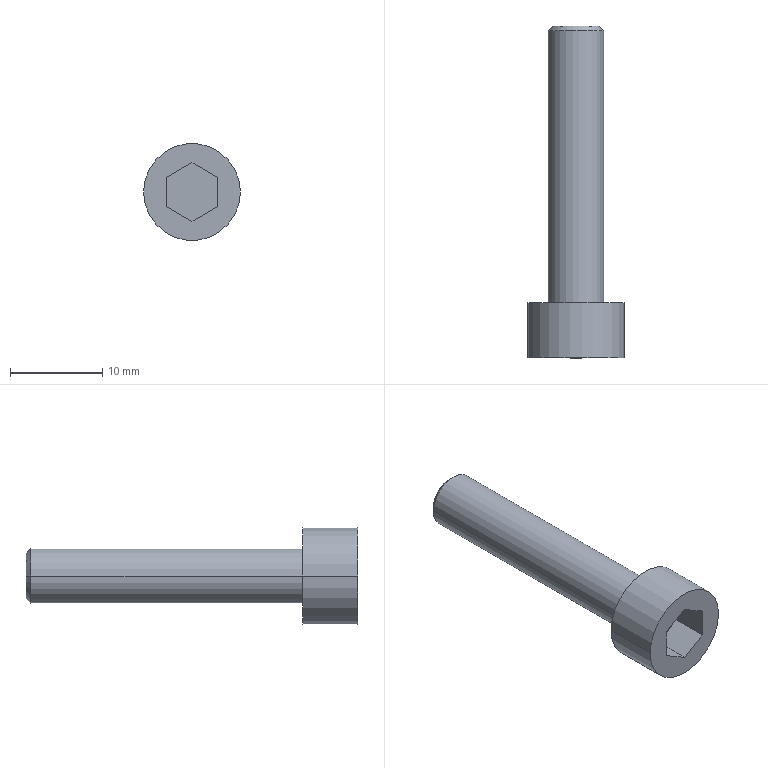Component | SolidWorks | M6x30HexSocketCap-1 | 1 solid | 16 faces | box 10.5 x 36 x 10.5 mm | volume 1261 mm3 | plane 10 | cylinder 4 | cone 2 | commonest cylinder face diameters 6 x2 10.5 x2 | material #45
build123d program:
from build123d import *

# Parameters (mm, degrees)
CUT_EXTRUDE1_DEPTH = 4


with BuildPart() as part:
    # Sketch1 → Revolve1 (revolve)
    with BuildSketch(Plane(origin=(0, 0, 0), x_dir=(1, 0, 0), z_dir=(0, 1, 0)), mode=Mode.PRIVATE) as revolve1_sk:
        Polygon((0, 36), (-5.25, 36), (-5.25, 30), (-3, 30), (-3, 0.5), (-2.5, 0), (0, 0), align=None)
    revolve(revolve1_sk.sketch.rotate(Axis((0, 0, 0), (0, 0, -1)), 180), axis=Axis((0, 0, 0), (0, 0, -1)))

    # Sketch2 → Cut-Extrude1 (cut)
    with BuildSketch(Plane(origin=(0, 0, -36), x_dir=(-1, 0, 0), z_dir=(0, 0, -1))):
        Polygon((0, 3.175), (-2.75, 1.588), (-2.75, -1.588), (0, -3.175), (2.75, -1.588), (2.75, 1.588), align=None)
    extrude(amount=-CUT_EXTRUDE1_DEPTH, mode=Mode.SUBTRACT)


solid = part.part

# Placed as in the assembly
solid = solid.moved(Location((-63, 340.7, 7.5), (-90, 0, 0)))
STEP:
#1=COLOUR_RGB('',0.7922,0.8196,0.9333);
#2=FILL_AREA_STYLE_COLOUR('',#1);
#3=FILL_AREA_STYLE('',(#2));
#4=SURFACE_STYLE_FILL_AREA(#3);
#5=SURFACE_SIDE_STYLE('',(#4));
#6=SURFACE_STYLE_USAGE(.BOTH.,#5);
#7=PRESENTATION_STYLE_ASSIGNMENT((#6));
#8=CARTESIAN_POINT('',(-2.382,13.413,0.2953));
#9=VERTEX_POINT('',#8);
#10=CARTESIAN_POINT('',(-2.579,13.413,0.2953));
#11=VERTEX_POINT('',#10);
#12=CARTESIAN_POINT('',(-2.48,13.413,0.2953));
#13=DIRECTION('',(0.,1.,-0.));
#14=DIRECTION('',(1.,0.,0.));
#15=AXIS2_PLACEMENT_3D('',#12,#13,#14);
#16=CIRCLE('',#15,0.09843);
#17=EDGE_CURVE('',#9,#11,#16,.T.);
#18=ORIENTED_EDGE('',*,*,#17,.F.);
#19=CARTESIAN_POINT('',(-2.362,13.394,0.2953));
#20=VERTEX_POINT('',#19);
#21=CARTESIAN_POINT('',(-2.362,13.394,0.2953));
#22=DIRECTION('',(0.7071,-0.7071,-0.));
#23=VECTOR('',#22,39.37);
#24=LINE('',#21,#23);
#25=EDGE_CURVE('',#9,#20,#24,.T.);
#26=ORIENTED_EDGE('',*,*,#25,.T.);
#27=CARTESIAN_POINT('',(-2.598,13.394,0.2953));
#28=VERTEX_POINT('',#27);
#29=CARTESIAN_POINT('',(-2.48,13.394,0.2953));
#30=DIRECTION('',(0.,1.,-0.));
#31=DIRECTION('',(1.,0.,0.));
#32=AXIS2_PLACEMENT_3D('',#29,#30,#31);
#33=CIRCLE('',#32,0.1181);
#34=EDGE_CURVE('',#20,#28,#33,.T.);
#35=ORIENTED_EDGE('',*,*,#34,.T.);
#36=CARTESIAN_POINT('',(-2.598,13.394,0.2953));
#37=DIRECTION('',(-0.7071,-0.7071,0.));
#38=VECTOR('',#37,39.37);
#39=LINE('',#36,#38);
#40=EDGE_CURVE('',#11,#28,#39,.T.);
#41=ORIENTED_EDGE('',*,*,#40,.F.);
#42=EDGE_LOOP('',(#18,#26,#35,#41));
#43=FACE_OUTER_BOUND('',#42,.T.);
#44=CARTESIAN_POINT('',(-2.48,13.394,0.2953));
#45=DIRECTION('',(-0.,-1.,0.));
#46=DIRECTION('',(-1.,0.,0.));
#47=AXIS2_PLACEMENT_3D('',#44,#45,#46);
#48=CONICAL_SURFACE('',#47,0.1181,0.7854);
#49=ADVANCED_FACE('',(#43),#48,.T.);
#50=CARTESIAN_POINT('',(-2.362,12.232,0.2953));
#51=VERTEX_POINT('',#50);
#52=CARTESIAN_POINT('',(-2.598,12.232,0.2953));
#53=VERTEX_POINT('',#52);
#54=CARTESIAN_POINT('',(-2.48,12.232,0.2953));
#55=DIRECTION('',(0.,1.,-0.));
#56=DIRECTION('',(1.,0.,0.));
#57=AXIS2_PLACEMENT_3D('',#54,#55,#56);
#58=CIRCLE('',#57,0.1181);
#59=EDGE_CURVE('',#51,#53,#58,.T.);
#60=ORIENTED_EDGE('',*,*,#59,.T.);
#61=CARTESIAN_POINT('',(-2.598,13.413,0.2953));
#62=DIRECTION('',(0.,1.,-0.));
#63=VECTOR('',#62,39.37);
#64=LINE('',#61,#63);
#65=EDGE_CURVE('',#53,#28,#64,.T.);
#66=ORIENTED_EDGE('',*,*,#65,.T.);
#67=ORIENTED_EDGE('',*,*,#34,.F.);
#68=CARTESIAN_POINT('',(-2.362,13.413,0.2953));
#69=DIRECTION('',(0.,1.,-0.));
#70=VECTOR('',#69,39.37);
#71=LINE('',#68,#70);
#72=EDGE_CURVE('',#51,#20,#71,.T.);
#73=ORIENTED_EDGE('',*,*,#72,.F.);
#74=EDGE_LOOP('',(#60,#66,#67,#73));
#75=FACE_OUTER_BOUND('',#74,.T.);
#76=CARTESIAN_POINT('',(-2.48,13.413,0.2953));
#77=DIRECTION('',(0.,1.,-0.));
#78=DIRECTION('',(1.,0.,0.));
#79=AXIS2_PLACEMENT_3D('',#76,#77,#78);
#80=CYLINDRICAL_SURFACE('',#79,0.1181);
#81=ADVANCED_FACE('',(#75),#80,.T.);
#82=CARTESIAN_POINT('',(-2.274,11.996,0.2953));
#83=VERTEX_POINT('',#82);
#84=CARTESIAN_POINT('',(-2.687,11.996,0.2953));
#85=VERTEX_POINT('',#84);
#86=CARTESIAN_POINT('',(-2.48,11.996,0.2953));
#87=DIRECTION('',(0.,1.,-0.));
#88=DIRECTION('',(1.,0.,0.));
#89=AXIS2_PLACEMENT_3D('',#86,#87,#88);
#90=CIRCLE('',#89,0.2067);
#91=EDGE_CURVE('',#83,#85,#90,.T.);
#92=ORIENTED_EDGE('',*,*,#91,.T.);
#93=CARTESIAN_POINT('',(-2.687,12.232,0.2953));
#94=VERTEX_POINT('',#93);
#95=CARTESIAN_POINT('',(-2.687,13.413,0.2953));
#96=DIRECTION('',(0.,1.,-0.));
#97=VECTOR('',#96,39.37);
#98=LINE('',#95,#97);
#99=EDGE_CURVE('',#85,#94,#98,.T.);
#100=ORIENTED_EDGE('',*,*,#99,.T.);
#101=CARTESIAN_POINT('',(-2.274,12.232,0.2953));
#102=VERTEX_POINT('',#101);
#103=CARTESIAN_POINT('',(-2.48,12.232,0.2953));
#104=DIRECTION('',(0.,1.,-0.));
#105=DIRECTION('',(1.,0.,0.));
#106=AXIS2_PLACEMENT_3D('',#103,#104,#105);
#107=CIRCLE('',#106,0.2067);
#108=EDGE_CURVE('',#102,#94,#107,.T.);
#109=ORIENTED_EDGE('',*,*,#108,.F.);
#110=CARTESIAN_POINT('',(-2.274,13.413,0.2953));
#111=DIRECTION('',(0.,1.,-0.));
#112=VECTOR('',#111,39.37);
#113=LINE('',#110,#112);
#114=EDGE_CURVE('',#83,#102,#113,.T.);
#115=ORIENTED_EDGE('',*,*,#114,.F.);
#116=EDGE_LOOP('',(#92,#100,#109,#115));
#117=FACE_OUTER_BOUND('',#116,.T.);
#118=CARTESIAN_POINT('',(-2.48,13.413,0.2953));
#119=DIRECTION('',(0.,1.,-0.));
#120=DIRECTION('',(1.,0.,0.));
#121=AXIS2_PLACEMENT_3D('',#118,#119,#120);
#122=CYLINDRICAL_SURFACE('',#121,0.2067);
#123=ADVANCED_FACE('',(#117),#122,.T.);
#124=CARTESIAN_POINT('',(-2.48,11.996,0.1703));
#125=VERTEX_POINT('',#124);
#126=CARTESIAN_POINT('',(-2.372,11.996,0.2328));
#127=VERTEX_POINT('',#126);
#128=CARTESIAN_POINT('',(-2.48,11.996,0.1703));
#129=DIRECTION('',(0.866,0.,0.5));
#130=VECTOR('',#129,39.37);
#131=LINE('',#128,#130);
#132=EDGE_CURVE('',#125,#127,#131,.T.);
#133=ORIENTED_EDGE('',*,*,#132,.F.);
#134=CARTESIAN_POINT('',(-2.589,11.996,0.2328));
#135=VERTEX_POINT('',#134);
#136=CARTESIAN_POINT('',(-2.589,11.996,0.2328));
#137=DIRECTION('',(0.866,-0.,-0.5));
#138=VECTOR('',#137,39.37);
#139=LINE('',#136,#138);
#140=EDGE_CURVE('',#135,#125,#139,.T.);
#141=ORIENTED_EDGE('',*,*,#140,.F.);
#142=CARTESIAN_POINT('',(-2.589,11.996,0.3578));
#143=VERTEX_POINT('',#142);
#144=CARTESIAN_POINT('',(-2.589,11.996,0.3578));
#145=DIRECTION('',(-0.,-0.,-1.));
#146=VECTOR('',#145,39.37);
#147=LINE('',#144,#146);
#148=EDGE_CURVE('',#143,#135,#147,.T.);
#149=ORIENTED_EDGE('',*,*,#148,.F.);
#150=CARTESIAN_POINT('',(-2.48,11.996,0.4203));
#151=VERTEX_POINT('',#150);
#152=CARTESIAN_POINT('',(-2.48,11.996,0.4203));
#153=DIRECTION('',(-0.866,-0.,-0.5));
#154=VECTOR('',#153,39.37);
#155=LINE('',#152,#154);
#156=EDGE_CURVE('',#151,#143,#155,.T.);
#157=ORIENTED_EDGE('',*,*,#156,.F.);
#158=CARTESIAN_POINT('',(-2.372,11.996,0.3578));
#159=VERTEX_POINT('',#158);
#160=CARTESIAN_POINT('',(-2.372,11.996,0.3578));
#161=DIRECTION('',(-0.866,0.,0.5));
#162=VECTOR('',#161,39.37);
#163=LINE('',#160,#162);
#164=EDGE_CURVE('',#159,#151,#163,.T.);
#165=ORIENTED_EDGE('',*,*,#164,.F.);
#166=CARTESIAN_POINT('',(-2.372,11.996,0.2328));
#167=DIRECTION('',(0.,0.,1.));
#168=VECTOR('',#167,39.37);
#169=LINE('',#166,#168);
#170=EDGE_CURVE('',#127,#159,#169,.T.);
#171=ORIENTED_EDGE('',*,*,#170,.F.);
#172=EDGE_LOOP('',(#133,#141,#149,#157,#165,#171));
#173=FACE_BOUND('',#172,.T.);
#174=ORIENTED_EDGE('',*,*,#91,.F.);
#175=CARTESIAN_POINT('',(-2.48,11.996,0.2953));
#176=DIRECTION('',(0.,1.,-0.));
#177=DIRECTION('',(1.,0.,0.));
#178=AXIS2_PLACEMENT_3D('',#175,#176,#177);
#179=CIRCLE('',#178,0.2067);
#180=EDGE_CURVE('',#85,#83,#179,.T.);
#181=ORIENTED_EDGE('',*,*,#180,.F.);
#182=EDGE_LOOP('',(#174,#181));
#183=FACE_OUTER_BOUND('',#182,.T.);
#184=CARTESIAN_POINT('',(-2.48,11.996,0.2953));
#185=DIRECTION('',(0.,1.,-0.));
#186=DIRECTION('',(1.,-0.,-0.));
#187=AXIS2_PLACEMENT_3D('',#184,#185,#186);
#188=PLANE('',#187);
#189=ADVANCED_FACE('',(#173,#183),#188,.F.);
#190=ORIENTED_EDGE('',*,*,#99,.F.);
#191=ORIENTED_EDGE('',*,*,#180,.T.);
#192=ORIENTED_EDGE('',*,*,#114,.T.);
#193=CARTESIAN_POINT('',(-2.48,12.232,0.2953));
#194=DIRECTION('',(0.,1.,-0.));
#195=DIRECTION('',(1.,0.,0.));
#196=AXIS2_PLACEMENT_3D('',#193,#194,#195);
#197=CIRCLE('',#196,0.2067);
#198=EDGE_CURVE('',#94,#102,#197,.T.);
#199=ORIENTED_EDGE('',*,*,#198,.F.);
#200=EDGE_LOOP('',(#190,#191,#192,#199));
#201=FACE_OUTER_BOUND('',#200,.T.);
#202=CARTESIAN_POINT('',(-2.48,13.413,0.2953));
#203=DIRECTION('',(0.,1.,-0.));
#204=DIRECTION('',(1.,0.,0.));
#205=AXIS2_PLACEMENT_3D('',#202,#203,#204);
#206=CYLINDRICAL_SURFACE('',#205,0.2067);
#207=ADVANCED_FACE('',(#201),#206,.T.);
#208=ORIENTED_EDGE('',*,*,#59,.F.);
#209=CARTESIAN_POINT('',(-2.48,12.232,0.2953));
#210=DIRECTION('',(0.,1.,-0.));
#211=DIRECTION('',(1.,0.,0.));
#212=AXIS2_PLACEMENT_3D('',#209,#210,#211);
#213=CIRCLE('',#212,0.1181);
#214=EDGE_CURVE('',#53,#51,#213,.T.);
#215=ORIENTED_EDGE('',*,*,#214,.F.);
#216=EDGE_LOOP('',(#208,#215));
#217=FACE_BOUND('',#216,.T.);
#218=ORIENTED_EDGE('',*,*,#108,.T.);
#219=ORIENTED_EDGE('',*,*,#198,.T.);
#220=EDGE_LOOP('',(#218,#219));
#221=FACE_OUTER_BOUND('',#220,.T.);
#222=CARTESIAN_POINT('',(-2.687,12.232,0.2953));
#223=DIRECTION('',(-0.,-1.,0.));
#224=DIRECTION('',(-1.,0.,0.));
#225=AXIS2_PLACEMENT_3D('',#222,#223,#224);
#226=PLANE('',#225);
#227=ADVANCED_FACE('',(#217,#221),#226,.F.);
#228=ORIENTED_EDGE('',*,*,#65,.F.);
#229=ORIENTED_EDGE('',*,*,#214,.T.);
#230=ORIENTED_EDGE('',*,*,#72,.T.);
#231=CARTESIAN_POINT('',(-2.48,13.394,0.2953));
#232=DIRECTION('',(0.,1.,-0.));
#233=DIRECTION('',(1.,0.,0.));
#234=AXIS2_PLACEMENT_3D('',#231,#232,#233);
#235=CIRCLE('',#234,0.1181);
#236=EDGE_CURVE('',#28,#20,#235,.T.);
#237=ORIENTED_EDGE('',*,*,#236,.F.);
#238=EDGE_LOOP('',(#228,#229,#230,#237));
#239=FACE_OUTER_BOUND('',#238,.T.);
#240=CARTESIAN_POINT('',(-2.48,13.413,0.2953));
#241=DIRECTION('',(0.,1.,-0.));
#242=DIRECTION('',(1.,0.,0.));
#243=AXIS2_PLACEMENT_3D('',#240,#241,#242);
#244=CYLINDRICAL_SURFACE('',#243,0.1181);
#245=ADVANCED_FACE('',(#239),#244,.T.);
#246=ORIENTED_EDGE('',*,*,#25,.F.);
#247=CARTESIAN_POINT('',(-2.48,13.413,0.2953));
#248=DIRECTION('',(0.,1.,-0.));
#249=DIRECTION('',(1.,0.,0.));
#250=AXIS2_PLACEMENT_3D('',#247,#248,#249);
#251=CIRCLE('',#250,0.09843);
#252=EDGE_CURVE('',#11,#9,#251,.T.);
#253=ORIENTED_EDGE('',*,*,#252,.F.);
#254=ORIENTED_EDGE('',*,*,#40,.T.);
#255=ORIENTED_EDGE('',*,*,#236,.T.);
#256=EDGE_LOOP('',(#246,#253,#254,#255));
#257=FACE_OUTER_BOUND('',#256,.T.);
#258=CARTESIAN_POINT('',(-2.48,13.394,0.2953));
#259=DIRECTION('',(-0.,-1.,0.));
#260=DIRECTION('',(-1.,0.,0.));
#261=AXIS2_PLACEMENT_3D('',#258,#259,#260);
#262=CONICAL_SURFACE('',#261,0.1181,0.7854);
#263=ADVANCED_FACE('',(#257),#262,.T.);
#264=ORIENTED_EDGE('',*,*,#252,.T.);
#265=ORIENTED_EDGE('',*,*,#17,.T.);
#266=EDGE_LOOP('',(#264,#265));
#267=FACE_OUTER_BOUND('',#266,.T.);
#268=CARTESIAN_POINT('',(-2.579,13.413,0.2953));
#269=DIRECTION('',(-0.,-1.,0.));
#270=DIRECTION('',(-1.,0.,0.));
#271=AXIS2_PLACEMENT_3D('',#268,#269,#270);
#272=PLANE('',#271);
#273=ADVANCED_FACE('',(#267),#272,.F.);
#274=ORIENTED_EDGE('',*,*,#140,.T.);
#275=CARTESIAN_POINT('',(-2.48,12.154,0.1703));
#276=VERTEX_POINT('',#275);
#277=CARTESIAN_POINT('',(-2.48,12.154,0.1703));
#278=DIRECTION('',(-0.,-1.,0.));
#279=VECTOR('',#278,39.37);
#280=LINE('',#277,#279);
#281=EDGE_CURVE('',#276,#125,#280,.T.);
#282=ORIENTED_EDGE('',*,*,#281,.F.);
#283=CARTESIAN_POINT('',(-2.589,12.154,0.2328));
#284=VERTEX_POINT('',#283);
#285=CARTESIAN_POINT('',(-2.589,12.154,0.2328));
#286=DIRECTION('',(0.866,-0.,-0.5));
#287=VECTOR('',#286,39.37);
#288=LINE('',#285,#287);
#289=EDGE_CURVE('',#284,#276,#288,.T.);
#290=ORIENTED_EDGE('',*,*,#289,.F.);
#291=CARTESIAN_POINT('',(-2.589,12.154,0.2328));
#292=DIRECTION('',(-0.,-1.,0.));
#293=VECTOR('',#292,39.37);
#294=LINE('',#291,#293);
#295=EDGE_CURVE('',#284,#135,#294,.T.);
#296=ORIENTED_EDGE('',*,*,#295,.T.);
#297=EDGE_LOOP('',(#274,#282,#290,#296));
#298=FACE_OUTER_BOUND('',#297,.T.);
#299=CARTESIAN_POINT('',(-2.589,12.154,0.2328));
#300=DIRECTION('',(-0.5,-0.,-0.866));
#301=DIRECTION('',(-0.866,0.,0.5));
#302=AXIS2_PLACEMENT_3D('',#299,#300,#301);
#303=PLANE('',#302);
#304=ADVANCED_FACE('',(#298),#303,.F.);
#305=ORIENTED_EDGE('',*,*,#148,.T.);
#306=ORIENTED_EDGE('',*,*,#295,.F.);
#307=CARTESIAN_POINT('',(-2.589,12.154,0.3578));
#308=VERTEX_POINT('',#307);
#309=CARTESIAN_POINT('',(-2.589,12.154,0.3578));
#310=DIRECTION('',(-0.,-0.,-1.));
#311=VECTOR('',#310,39.37);
#312=LINE('',#309,#311);
#313=EDGE_CURVE('',#308,#284,#312,.T.);
#314=ORIENTED_EDGE('',*,*,#313,.F.);
#315=CARTESIAN_POINT('',(-2.589,12.154,0.3578));
#316=DIRECTION('',(-0.,-1.,0.));
#317=VECTOR('',#316,39.37);
#318=LINE('',#315,#317);
#319=EDGE_CURVE('',#308,#143,#318,.T.);
#320=ORIENTED_EDGE('',*,*,#319,.T.);
#321=EDGE_LOOP('',(#305,#306,#314,#320));
#322=FACE_OUTER_BOUND('',#321,.T.);
#323=CARTESIAN_POINT('',(-2.589,12.154,0.3578));
#324=DIRECTION('',(-1.,0.,0.));
#325=DIRECTION('',(0.,1.,-0.));
#326=AXIS2_PLACEMENT_3D('',#323,#324,#325);
#327=PLANE('',#326);
#328=ADVANCED_FACE('',(#322),#327,.F.);
#329=ORIENTED_EDGE('',*,*,#156,.T.);
#330=ORIENTED_EDGE('',*,*,#319,.F.);
#331=CARTESIAN_POINT('',(-2.48,12.154,0.4203));
#332=VERTEX_POINT('',#331);
#333=CARTESIAN_POINT('',(-2.48,12.154,0.4203));
#334=DIRECTION('',(-0.866,-0.,-0.5));
#335=VECTOR('',#334,39.37);
#336=LINE('',#333,#335);
#337=EDGE_CURVE('',#332,#308,#336,.T.);
#338=ORIENTED_EDGE('',*,*,#337,.F.);
#339=CARTESIAN_POINT('',(-2.48,12.154,0.4203));
#340=DIRECTION('',(-0.,-1.,0.));
#341=VECTOR('',#340,39.37);
#342=LINE('',#339,#341);
#343=EDGE_CURVE('',#332,#151,#342,.T.);
#344=ORIENTED_EDGE('',*,*,#343,.T.);
#345=EDGE_LOOP('',(#329,#330,#338,#344));
#346=FACE_OUTER_BOUND('',#345,.T.);
#347=CARTESIAN_POINT('',(-2.48,12.154,0.4203));
#348=DIRECTION('',(-0.5,0.,0.866));
#349=DIRECTION('',(0.866,0.,0.5));
#350=AXIS2_PLACEMENT_3D('',#347,#348,#349);
#351=PLANE('',#350);
#352=ADVANCED_FACE('',(#346),#351,.F.);
#353=ORIENTED_EDGE('',*,*,#164,.T.);
#354=ORIENTED_EDGE('',*,*,#343,.F.);
#355=CARTESIAN_POINT('',(-2.372,12.154,0.3578));
#356=VERTEX_POINT('',#355);
#357=CARTESIAN_POINT('',(-2.372,12.154,0.3578));
#358=DIRECTION('',(-0.866,0.,0.5));
#359=VECTOR('',#358,39.37);
#360=LINE('',#357,#359);
#361=EDGE_CURVE('',#356,#332,#360,.T.);
#362=ORIENTED_EDGE('',*,*,#361,.F.);
#363=CARTESIAN_POINT('',(-2.372,12.154,0.3578));
#364=DIRECTION('',(-0.,-1.,0.));
#365=VECTOR('',#364,39.37);
#366=LINE('',#363,#365);
#367=EDGE_CURVE('',#356,#159,#366,.T.);
#368=ORIENTED_EDGE('',*,*,#367,.T.);
#369=EDGE_LOOP('',(#353,#354,#362,#368));
#370=FACE_OUTER_BOUND('',#369,.T.);
#371=CARTESIAN_POINT('',(-2.372,12.154,0.3578));
#372=DIRECTION('',(0.5,0.,0.866));
#373=DIRECTION('',(0.866,-0.,-0.5));
#374=AXIS2_PLACEMENT_3D('',#371,#372,#373);
#375=PLANE('',#374);
#376=ADVANCED_FACE('',(#370),#375,.F.);
#377=ORIENTED_EDGE('',*,*,#170,.T.);
#378=ORIENTED_EDGE('',*,*,#367,.F.);
#379=CARTESIAN_POINT('',(-2.372,12.154,0.2328));
#380=VERTEX_POINT('',#379);
#381=CARTESIAN_POINT('',(-2.372,12.154,0.2328));
#382=DIRECTION('',(0.,0.,1.));
#383=VECTOR('',#382,39.37);
#384=LINE('',#381,#383);
#385=EDGE_CURVE('',#380,#356,#384,.T.);
#386=ORIENTED_EDGE('',*,*,#385,.F.);
#387=CARTESIAN_POINT('',(-2.372,12.154,0.2328));
#388=DIRECTION('',(-0.,-1.,0.));
#389=VECTOR('',#388,39.37);
#390=LINE('',#387,#389);
#391=EDGE_CURVE('',#380,#127,#390,.T.);
#392=ORIENTED_EDGE('',*,*,#391,.T.);
#393=EDGE_LOOP('',(#377,#378,#386,#392));
#394=FACE_OUTER_BOUND('',#393,.T.);
#395=CARTESIAN_POINT('',(-2.372,12.154,0.2328));
#396=DIRECTION('',(1.,-0.,-0.));
#397=DIRECTION('',(-0.,-1.,0.));
#398=AXIS2_PLACEMENT_3D('',#395,#396,#397);
#399=PLANE('',#398);
#400=ADVANCED_FACE('',(#394),#399,.F.);
#401=ORIENTED_EDGE('',*,*,#132,.T.);
#402=ORIENTED_EDGE('',*,*,#391,.F.);
#403=CARTESIAN_POINT('',(-2.48,12.154,0.1703));
#404=DIRECTION('',(0.866,0.,0.5));
#405=VECTOR('',#404,39.37);
#406=LINE('',#403,#405);
#407=EDGE_CURVE('',#276,#380,#406,.T.);
#408=ORIENTED_EDGE('',*,*,#407,.F.);
#409=ORIENTED_EDGE('',*,*,#281,.T.);
#410=EDGE_LOOP('',(#401,#402,#408,#409));
#411=FACE_OUTER_BOUND('',#410,.T.);
#412=CARTESIAN_POINT('',(-2.48,12.154,0.1703));
#413=DIRECTION('',(0.5,-0.,-0.866));
#414=DIRECTION('',(-0.866,-0.,-0.5));
#415=AXIS2_PLACEMENT_3D('',#412,#413,#414);
#416=PLANE('',#415);
#417=ADVANCED_FACE('',(#411),#416,.F.);
#418=ORIENTED_EDGE('',*,*,#289,.T.);
#419=ORIENTED_EDGE('',*,*,#407,.T.);
#420=ORIENTED_EDGE('',*,*,#385,.T.);
#421=ORIENTED_EDGE('',*,*,#361,.T.);
#422=ORIENTED_EDGE('',*,*,#337,.T.);
#423=ORIENTED_EDGE('',*,*,#313,.T.);
#424=EDGE_LOOP('',(#418,#419,#420,#421,#422,#423));
#425=FACE_OUTER_BOUND('',#424,.T.);
#426=CARTESIAN_POINT('',(-2.48,12.154,0.2953));
#427=DIRECTION('',(-0.,-1.,0.));
#428=DIRECTION('',(-1.,0.,0.));
#429=AXIS2_PLACEMENT_3D('',#426,#427,#428);
#430=PLANE('',#429);
#431=ADVANCED_FACE('',(#425),#430,.T.);
#432=CLOSED_SHELL('',(#49,#81,#123,#189,#207,#227,#245,#263,#273,#304,#328,#352,#376,#400,#417,#431));
#433=MANIFOLD_SOLID_BREP('',#432);
#434=STYLED_ITEM('',(#7),#433);
#435=PRESENTATION_LAYER_ASSIGNMENT('','',(#434));
#436=(LENGTH_UNIT()NAMED_UNIT(*)SI_UNIT($,.METRE.));
#437=LENGTH_MEASURE_WITH_UNIT(LENGTH_MEASURE(0.0254),#436);
#438=DIMENSIONAL_EXPONENTS(1.,0.,0.,0.,0.,0.,0.);
#439=(CONVERSION_BASED_UNIT('',#437)LENGTH_UNIT()NAMED_UNIT(#438));
#440=UNCERTAINTY_MEASURE_WITH_UNIT(LENGTH_MEASURE(0.00001),#439,'','');
#441=(NAMED_UNIT(*)PLANE_ANGLE_UNIT()SI_UNIT($,.RADIAN.));
#442=(NAMED_UNIT(*)SI_UNIT($,.STERADIAN.)SOLID_ANGLE_UNIT());
#443=(GEOMETRIC_REPRESENTATION_CONTEXT(3)GLOBAL_UNCERTAINTY_ASSIGNED_CONTEXT((#440))GLOBAL_UNIT_ASSIGNED_CONTEXT((#439,#441,#442))REPRESENTATION_CONTEXT('',''));
#444=MECHANICAL_DESIGN_GEOMETRIC_PRESENTATION_REPRESENTATION('',(#434),#443);
#445=CARTESIAN_POINT('',(0.,0.,0.));
#446=DIRECTION('',(0.,0.,1.));
#447=DIRECTION('',(1.,0.,0.));
#448=AXIS2_PLACEMENT_3D('',#445,#446,#447);
#449=(LENGTH_UNIT()NAMED_UNIT(*)SI_UNIT($,.METRE.));
#450=LENGTH_MEASURE_WITH_UNIT(LENGTH_MEASURE(0.0254),#449);
#451=DIMENSIONAL_EXPONENTS(1.,0.,0.,0.,0.,0.,0.);
#452=(CONVERSION_BASED_UNIT('',#450)LENGTH_UNIT()NAMED_UNIT(#451));
#453=UNCERTAINTY_MEASURE_WITH_UNIT(LENGTH_MEASURE(0.00001),#452,'','');
#454=(NAMED_UNIT(*)PLANE_ANGLE_UNIT()SI_UNIT($,.RADIAN.));
#455=(NAMED_UNIT(*)SI_UNIT($,.STERADIAN.)SOLID_ANGLE_UNIT());
#456=(GEOMETRIC_REPRESENTATION_CONTEXT(3)GLOBAL_UNCERTAINTY_ASSIGNED_CONTEXT((#453))GLOBAL_UNIT_ASSIGNED_CONTEXT((#452,#454,#455))REPRESENTATION_CONTEXT('',''));
#457=ADVANCED_BREP_SHAPE_REPRESENTATION('',(#433,#448),#456);